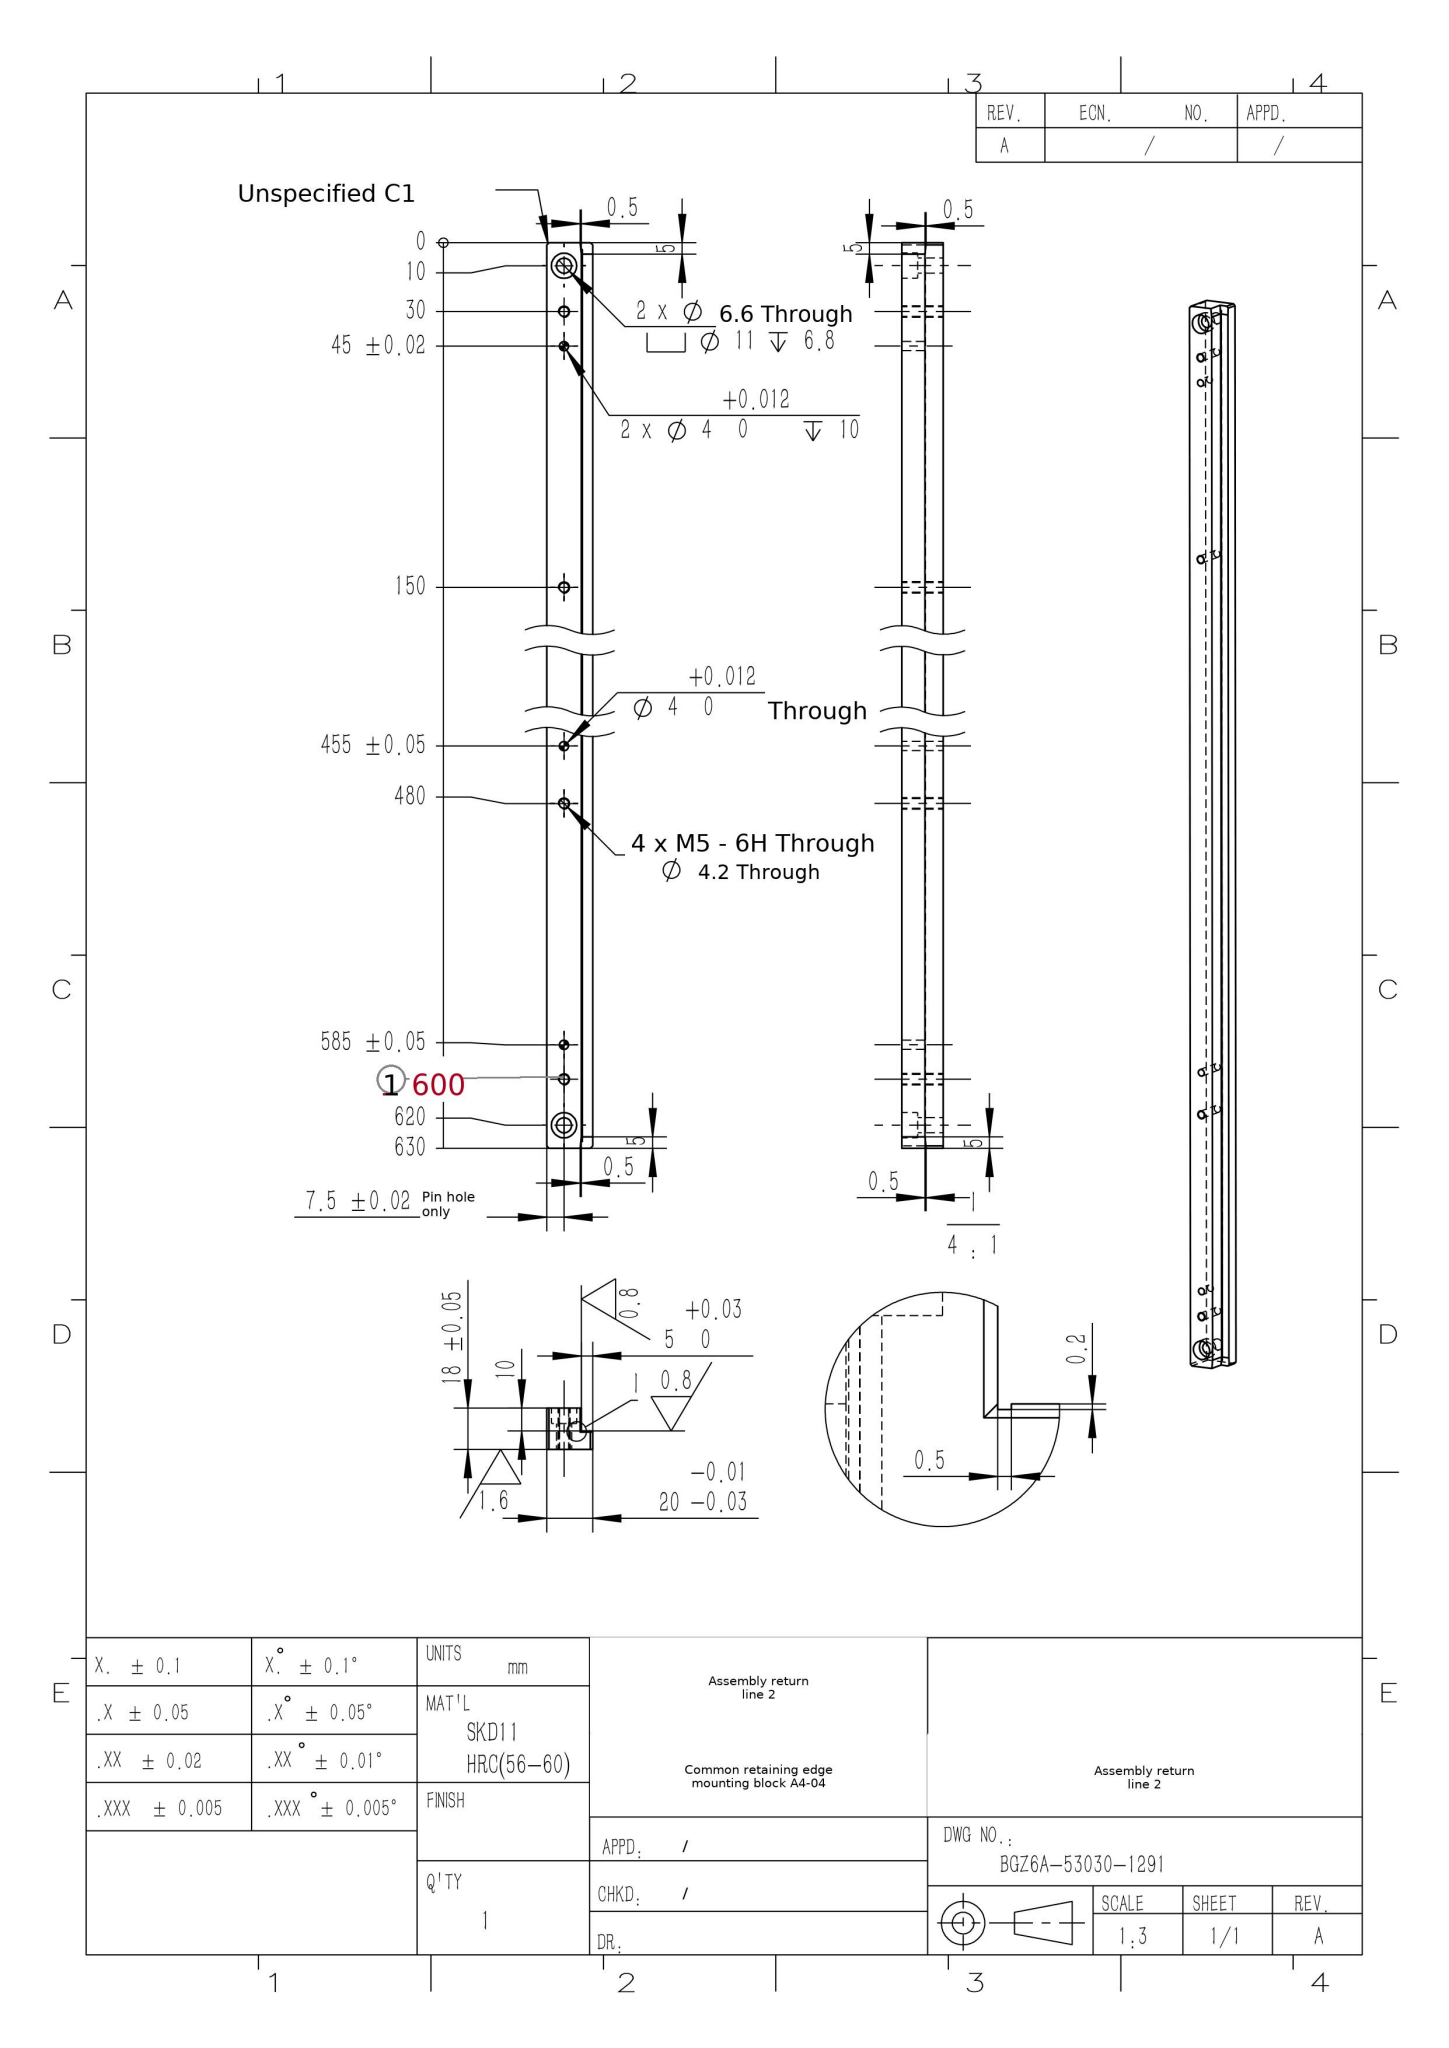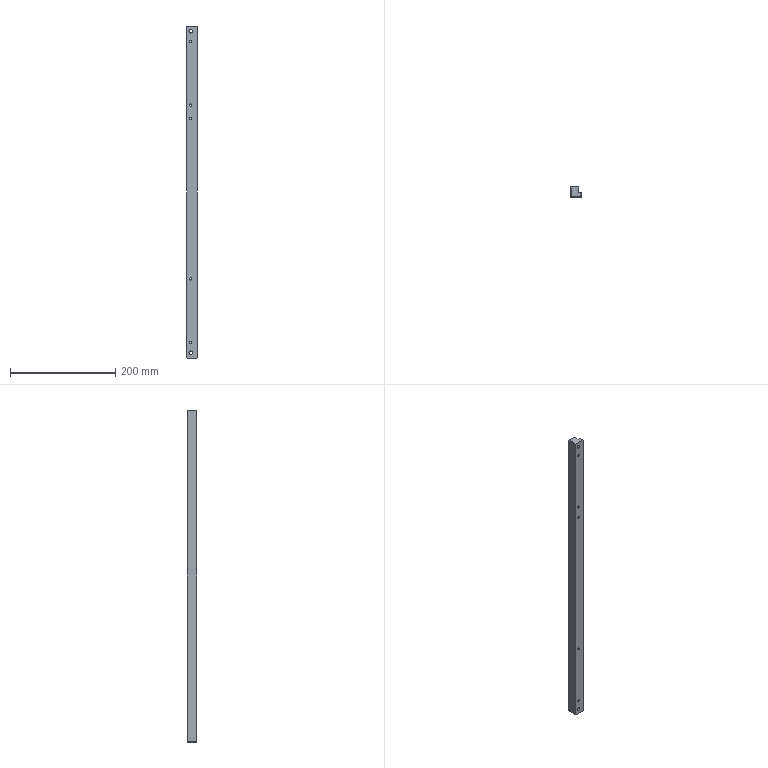Part | SolidWorks | mm | material SKD11 | 1 solid | 44 faces | box 20 x 18 x 630 mm | volume 191640 mm3 | cylinder 22 | plane 22 | commonest cylinder face diameters 4.2 x8 4 x6 11 x4 6.6 x4
build123d program:
from build123d import *
from OCP.BRepFilletAPI import BRepFilletAPI_MakeChamfer

# Parameters (mm, degrees)
BOSS_EXTRUDE1_DEPTH                             = 630
CHAMFER1_SIZE                                   = 0.5
CHAMFER1_SIZE2                                  = 5.001
SKETCH2_W                                       = 0.5
SKETCH2_H                                       = 0.2
CUT_EXTRUDE1_DEPTH                              = 631.574
CHAMFER2_SIZE                                   = 1
F_4_0_MM_DOWEL_PIN_HOLE_1_D                     = 4
F_4_0_MM_DOWEL_PIN_HOLE_1_DEPTH                 = 10
M5_TAPPED_HOLE2_D                               = 4.2
M6_HEX_SOCKET_HEAD_CAP_SCREW_CBORE1_D           = 6.6
M6_HEX_SOCKET_HEAD_CAP_SCREW_CBORE1_CBORE_D     = 11
M6_HEX_SOCKET_HEAD_CAP_SCREW_CBORE1_CBORE_DEPTH = 6.8
F_4_0MM_DOWEL_PIN_HOLE_3_D                      = 4


with BuildPart() as part:
    # Sketch1 → Boss-Extrude1 (new body)
    with BuildSketch(Plane.XY):
        Polygon((0, 0), (0, 18), (15, 18), (15, 8), (20, 8), (20, 0), align=None)
    extrude(amount=BOSS_EXTRUDE1_DEPTH)

    # Chamfer1: one chamfer whose edges measure the first distance from different faces: ONE call of the kernel's chamfer builder (chamfer() names one face for all edges)
    chamfer1_edges_1 = [part.edges().sort_by_distance(p)[0] for p in [
        (17.5, 8, 630),
        (15, 13, 630),
    ]]
    chamfer1_side_1 = [part.faces().sort_by_distance(p)[0] for p in [
        (8.79, 8.355, 630),
    ]]
    chamfer1_edges_2 = [part.edges().sort_by_distance(p)[0] for p in [
        (15, 13, 0),
        (17.5, 8, 0),
    ]]
    chamfer1_side_2 = [part.faces().sort_by_distance(p)[0] for p in [
        (8.79, 8.355, 0),
    ]]
    chamfer1 = BRepFilletAPI_MakeChamfer(part.part.solid().wrapped)
    for e in chamfer1_edges_1:
        chamfer1.Add(CHAMFER1_SIZE, CHAMFER1_SIZE2, e.wrapped, chamfer1_side_1[0].wrapped)  # the first distance lies on this face
    for e in chamfer1_edges_2:
        chamfer1.Add(CHAMFER1_SIZE, CHAMFER1_SIZE2, e.wrapped, chamfer1_side_2[0].wrapped)  # the first distance lies on this face
    add(Compound.cast(chamfer1.Shape()), mode=Mode.REPLACE)

    # Sketch2 → Cut-Extrude1 (cut, through all)
    with BuildSketch(Plane.XY.offset(630)):
        with Locations((15.25, 7.9)):
            Rectangle(SKETCH2_W, SKETCH2_H)
    extrude(amount=-CUT_EXTRUDE1_DEPTH, mode=Mode.SUBTRACT)

    # Chamfer2
    chamfer2_edges = [part.edges().sort_by_distance(p)[0] for p in [
        (0, 9, 630),
        (0, 9, 0),
        (20, 3.75, 0),
        (20, 3.75, 630),
    ]]
    chamfer(chamfer2_edges, length=CHAMFER2_SIZE)

    # 4.0 mm Dowel Pin Hole 1
    with Locations(Plane(origin=(0, 18, 0), x_dir=(1, 0, 0), z_dir=(0, 1, 0))):
        with Locations((7.5, -45), (7.5, -585)):
            Hole(F_4_0_MM_DOWEL_PIN_HOLE_1_D / 2, depth=F_4_0_MM_DOWEL_PIN_HOLE_1_DEPTH)

    # M5 Tapped Hole2 (through all)
    with Locations(Plane(origin=(0, 18, 0), x_dir=(1, 0, 0), z_dir=(0, 1, 0))):
        with Locations((7.5, -480), (7.5, -150), (7.5, -30), (7.5, -600)):
            Hole(M5_TAPPED_HOLE2_D / 2)

    # M6 Hex Socket Head Cap Screw CBORE1 (through all)
    with Locations(Plane(origin=(0, 18, 0), x_dir=(1, 0, 0), z_dir=(0, 1, 0))):
        with Locations((7.5, -620), (7.5, -10)):
            CounterBoreHole(M6_HEX_SOCKET_HEAD_CAP_SCREW_CBORE1_D / 2, M6_HEX_SOCKET_HEAD_CAP_SCREW_CBORE1_CBORE_D / 2, M6_HEX_SOCKET_HEAD_CAP_SCREW_CBORE1_CBORE_DEPTH)

    # 4.0mm Dowel Pin Hole 3 (through all)
    with Locations(Plane(origin=(0, 18, 0), x_dir=(1, 0, 0), z_dir=(0, 1, 0))):
        with Locations((7.5, -455)):
            Hole(F_4_0MM_DOWEL_PIN_HOLE_3_D / 2)


solid = part.part